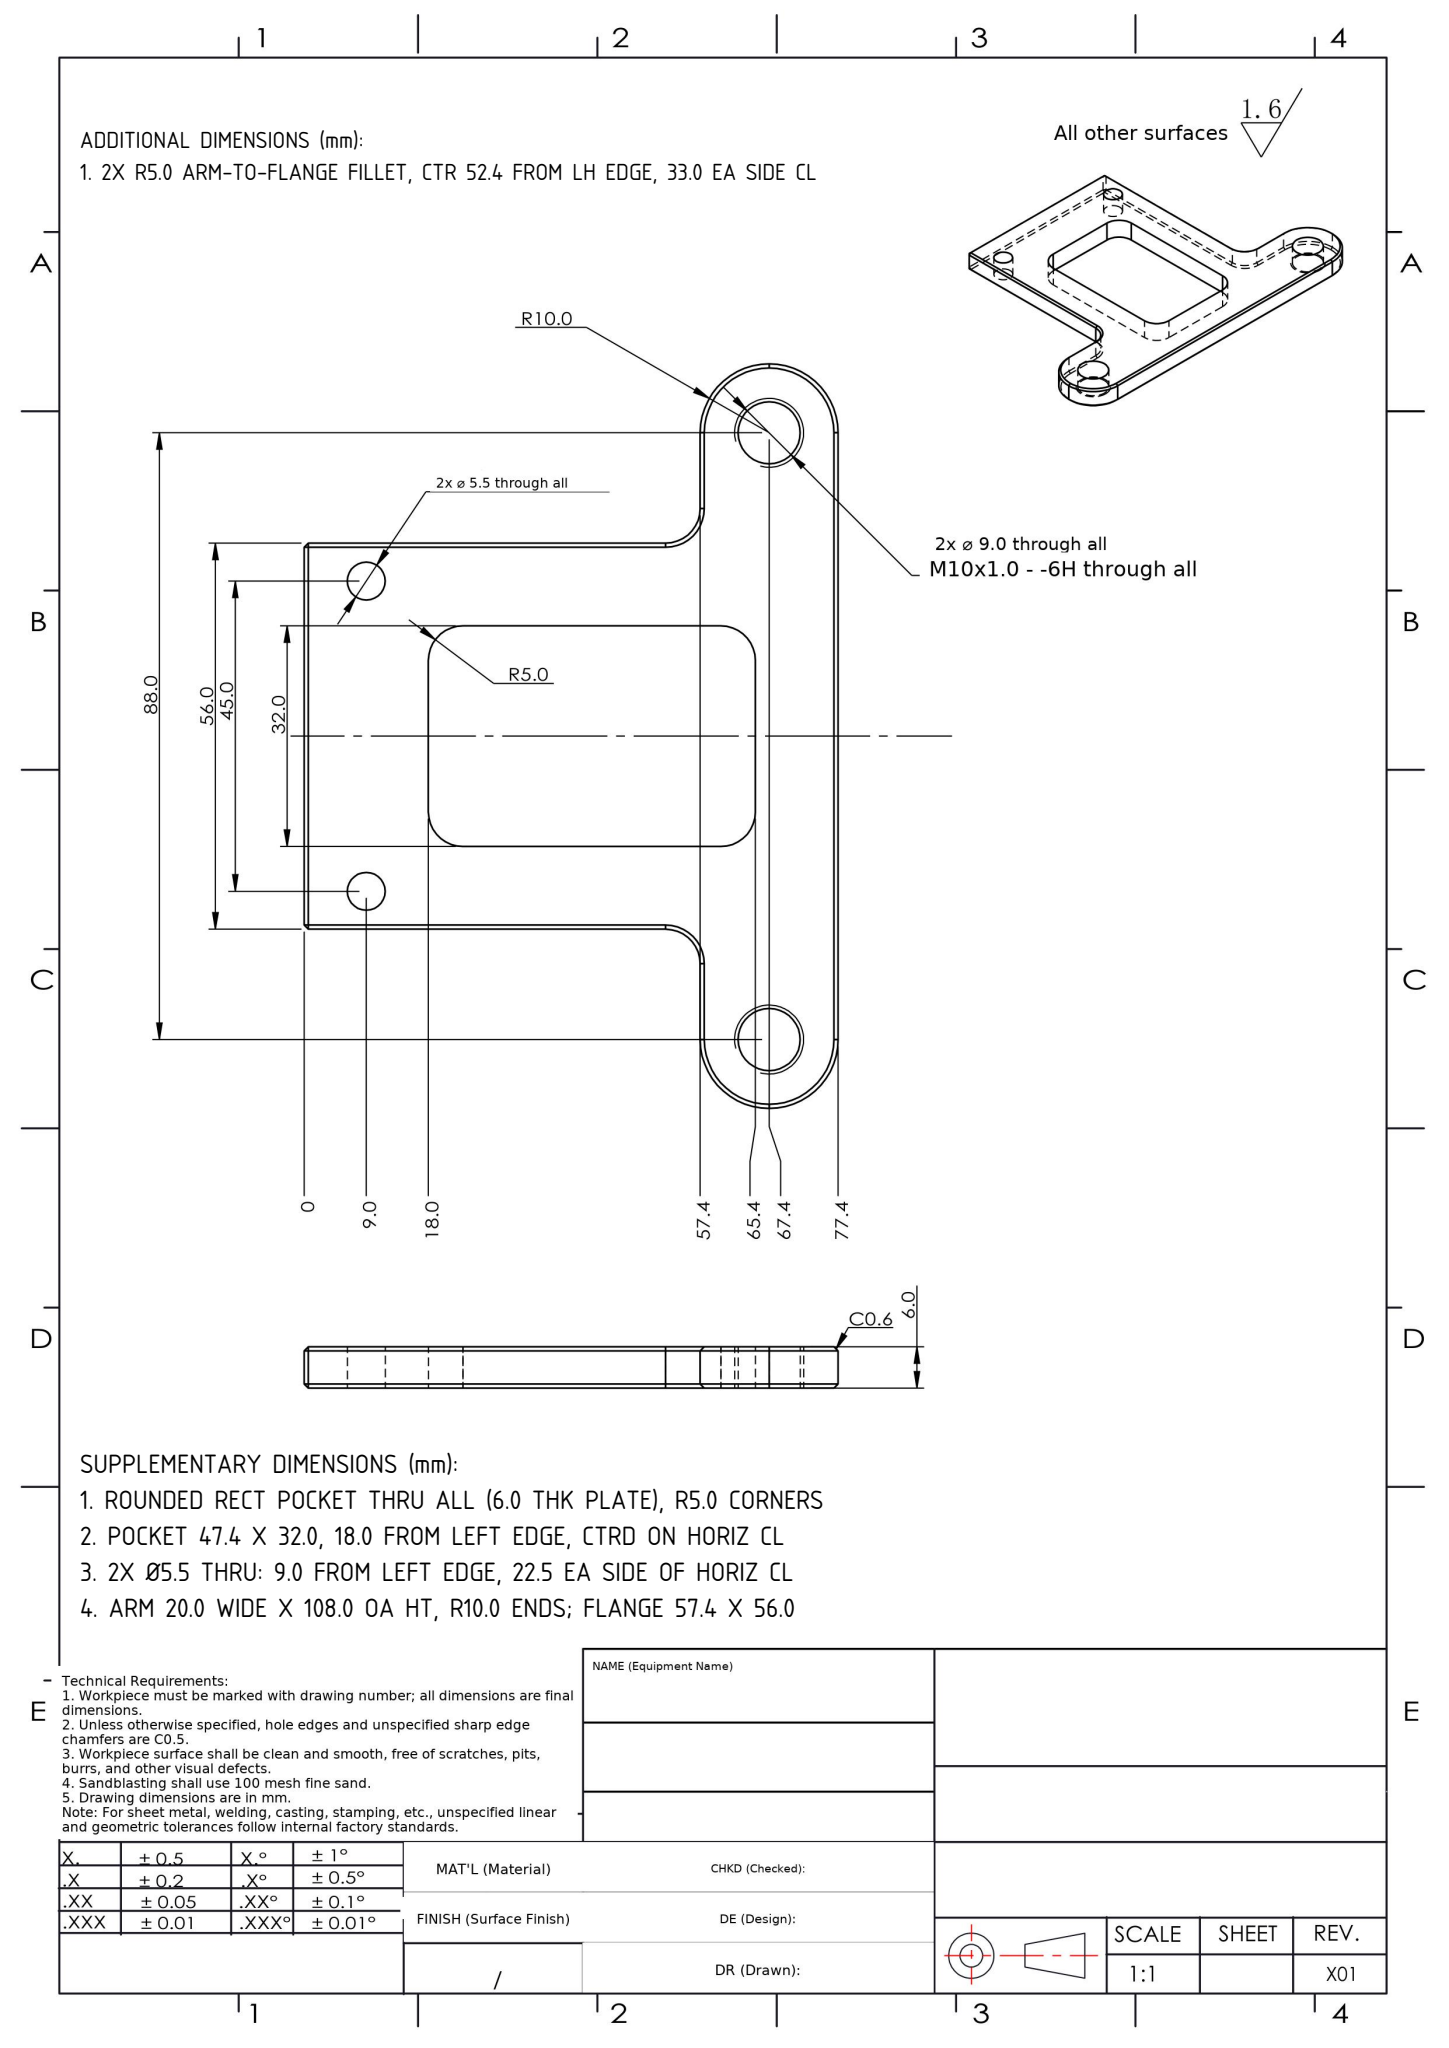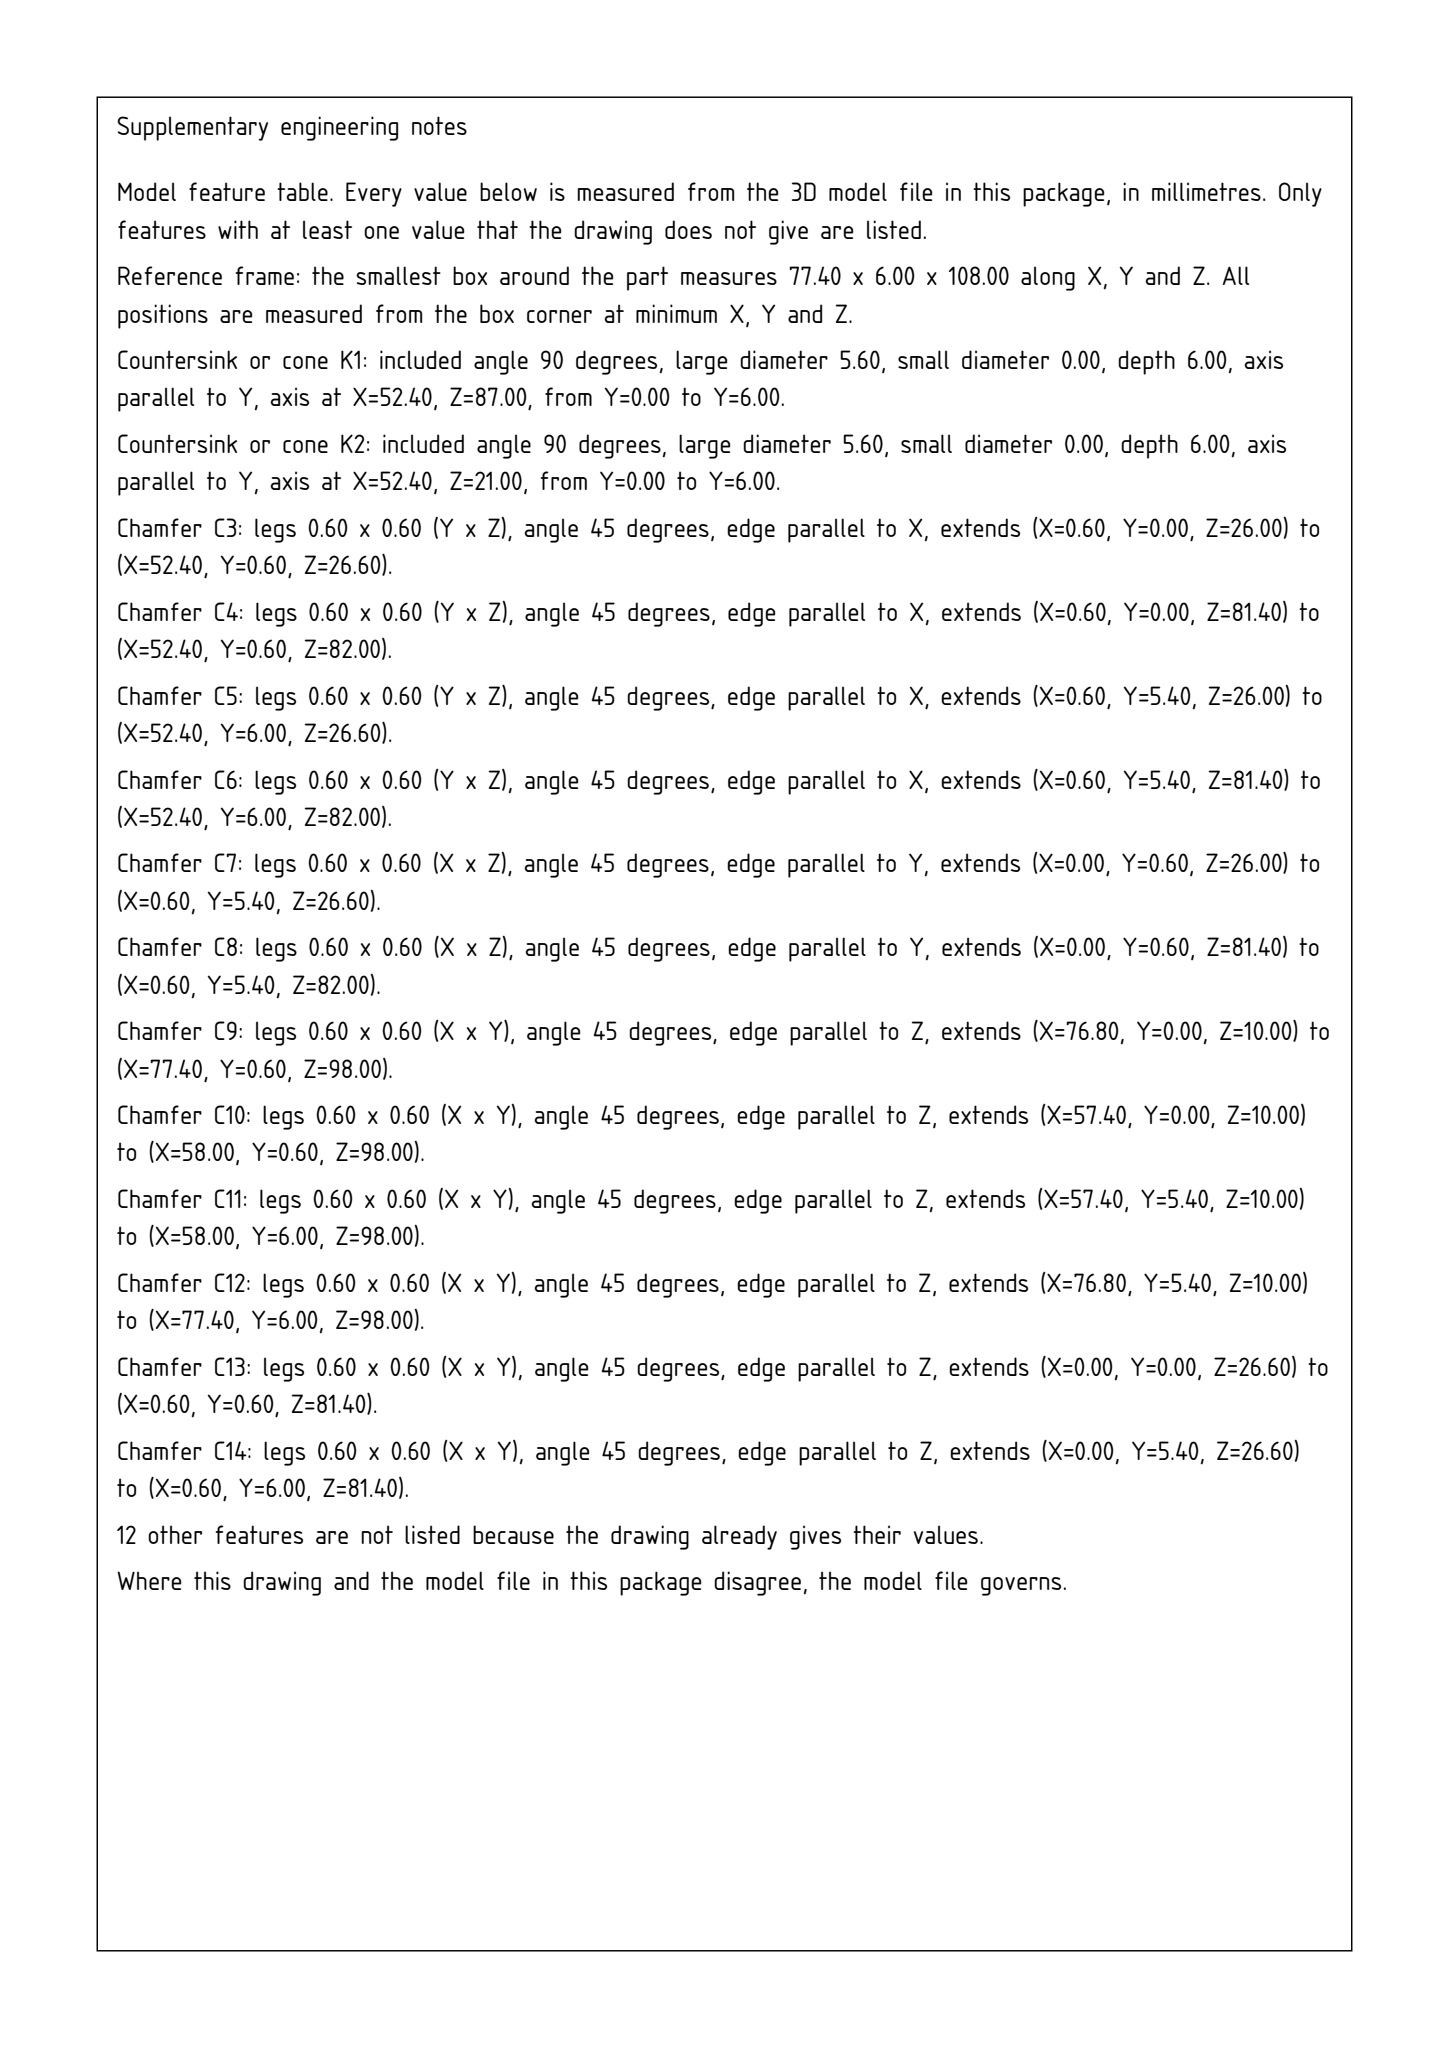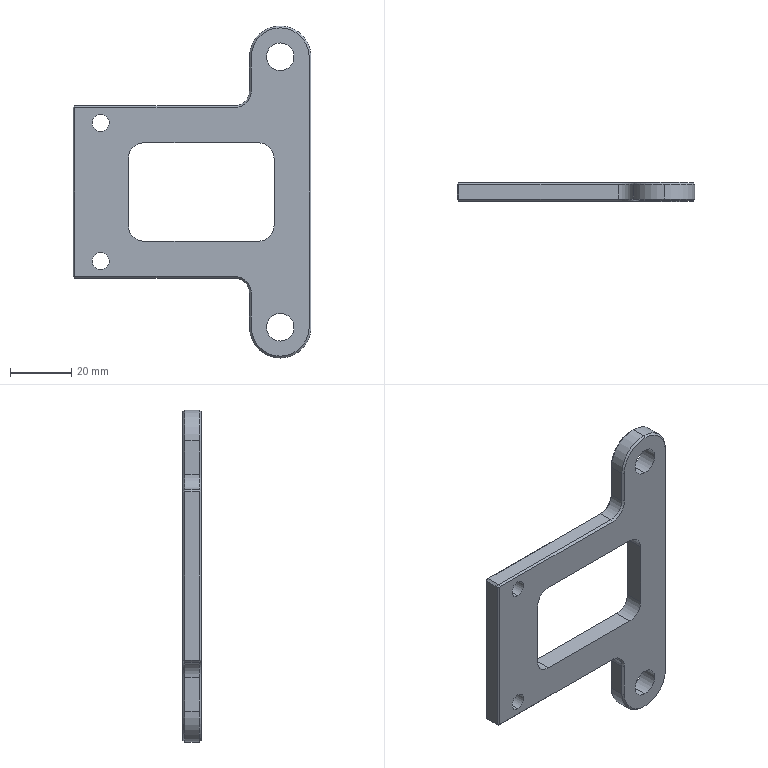Part | SolidWorks | mm | 1 solid | 60 faces | box 77.4 x 6 x 108 mm | volume 21648 mm3 | plane 30 | cylinder 18 | cone 12 | commonest cylinder face diameters 10 x6 9 x4 5.5 x4 20 x4